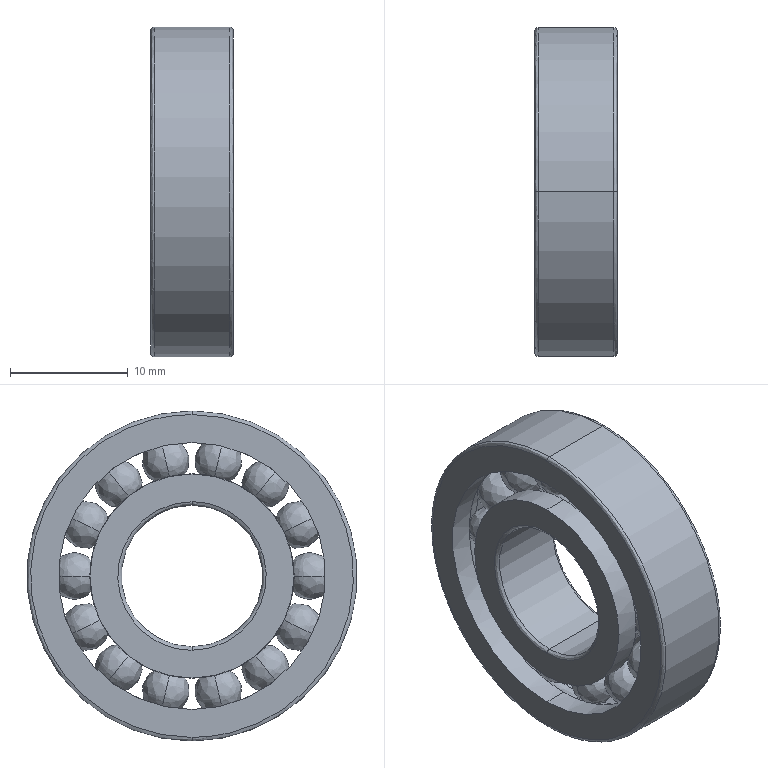Component | SolidWorks | ClampingAssembly-1_DeepGrooveBallBearing16001-1 | 1 solid | 97 faces | volume 2641 mm3 | spline 81 | cylinder 12 | plane 4 | commonest cylinder face diameters 22.667 x4 17.333 x4 28 x2 12 x2 | material Standard Part